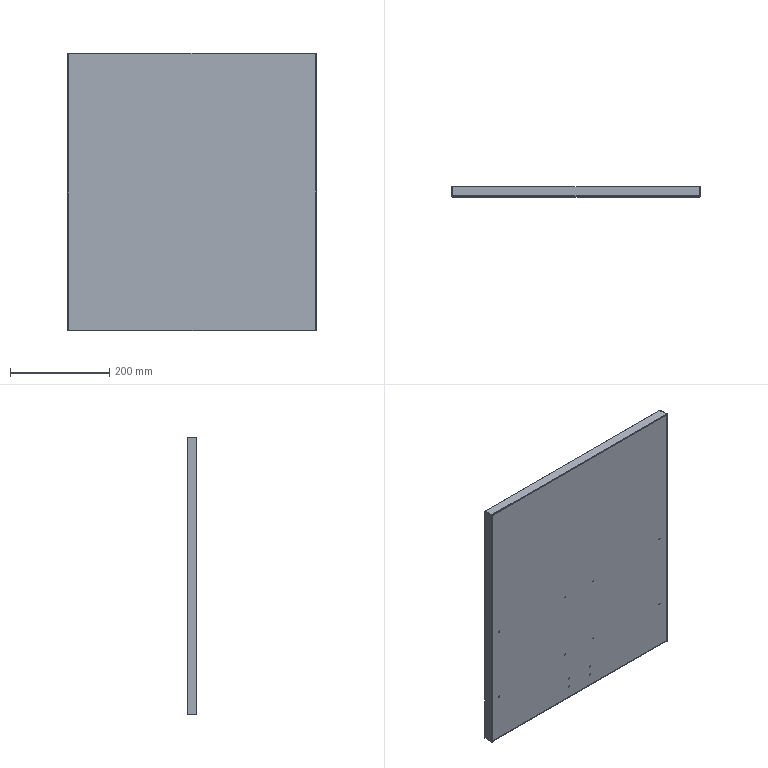Component | SolidWorks | BottomPlateWelding-2_BottomPlate-1 | 1 solid | 78 faces | volume 479004 mm3 | plane 46 | cylinder 32 | commonest cylinder face diameters 4 x24 3.2 x4 0.2 x4